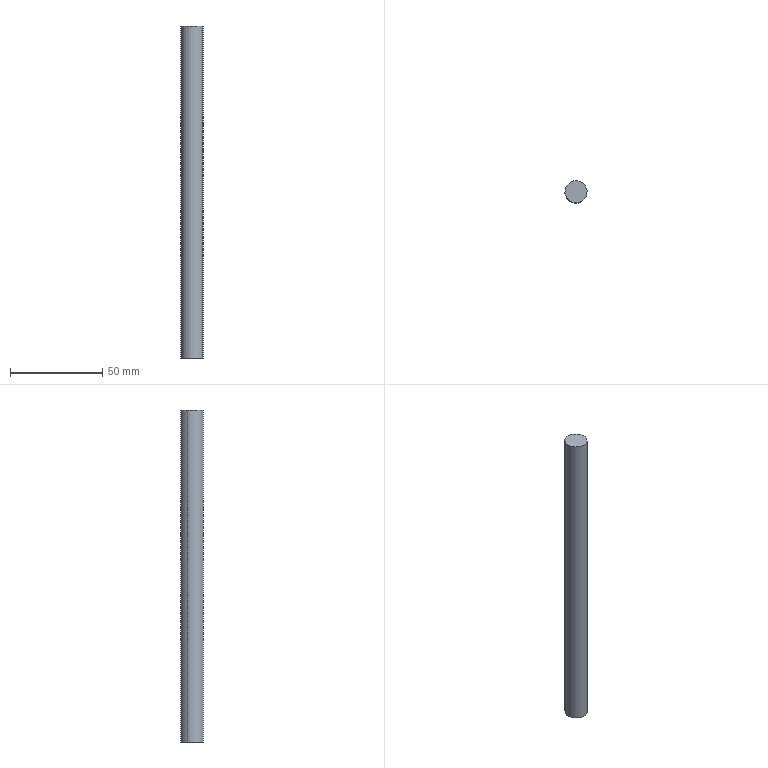Component | SolidWorks | MainAxis-1 | 1 solid | 4 faces | box 12 x 12 x 180 mm | volume 20358 mm3 | cylinder 2 | plane 2 | commonest cylinder face diameters 12 x2
build123d program:
from build123d import *

# Parameters (mm, degrees)
BOSS_EXTRUDE1_DEPTH      = 100
BOSS_EXTRUDE1_DEPTH_BACK = 80
SKETCH1_R                = 6


with BuildPart() as part:
    # Sketch1 → Boss-Extrude1 (new, two sides: drawn at the far end of the back side and taken through both)
    with BuildSketch(Plane.XY.offset(-BOSS_EXTRUDE1_DEPTH_BACK)):
        with Locations((-45, 0)):
            Circle(SKETCH1_R)
    extrude(amount=BOSS_EXTRUDE1_DEPTH + BOSS_EXTRUDE1_DEPTH_BACK)


solid = part.part

# Placed as in the assembly
solid = solid.moved(Location((-24.375, -67.172, 27.182), (0, 0, 0)))
STEP:
#1=CARTESIAN_POINT('',(-2.948,-2.551,-2.079));
#2=VERTEX_POINT('',#1);
#3=CARTESIAN_POINT('',(-2.514,-2.738,-2.079));
#4=VERTEX_POINT('',#3);
#5=CARTESIAN_POINT('',(-2.731,-2.645,-2.079));
#6=DIRECTION('',(-0.,0.,1.));
#7=DIRECTION('',(-0.918,0.3966,0.));
#8=AXIS2_PLACEMENT_3D('',#5,#6,#7);
#9=CIRCLE('',#8,0.2362);
#10=EDGE_CURVE('',#2,#4,#9,.T.);
#11=ORIENTED_EDGE('',*,*,#10,.T.);
#12=CARTESIAN_POINT('',(-2.514,-2.738,5.007));
#13=VERTEX_POINT('',#12);
#14=CARTESIAN_POINT('',(-2.514,-2.738,-2.079));
#15=DIRECTION('',(-0.,0.,1.));
#16=VECTOR('',#15,39.37);
#17=LINE('',#14,#16);
#18=EDGE_CURVE('',#4,#13,#17,.T.);
#19=ORIENTED_EDGE('',*,*,#18,.T.);
#20=CARTESIAN_POINT('',(-2.948,-2.551,5.007));
#21=VERTEX_POINT('',#20);
#22=CARTESIAN_POINT('',(-2.731,-2.645,5.007));
#23=DIRECTION('',(-0.,0.,1.));
#24=DIRECTION('',(-0.918,0.3966,0.));
#25=AXIS2_PLACEMENT_3D('',#22,#23,#24);
#26=CIRCLE('',#25,0.2362);
#27=EDGE_CURVE('',#21,#13,#26,.T.);
#28=ORIENTED_EDGE('',*,*,#27,.F.);
#29=CARTESIAN_POINT('',(-2.948,-2.551,-2.079));
#30=DIRECTION('',(-0.,0.,1.));
#31=VECTOR('',#30,39.37);
#32=LINE('',#29,#31);
#33=EDGE_CURVE('',#2,#21,#32,.T.);
#34=ORIENTED_EDGE('',*,*,#33,.F.);
#35=EDGE_LOOP('',(#11,#19,#28,#34));
#36=FACE_OUTER_BOUND('',#35,.T.);
#37=CARTESIAN_POINT('',(-2.731,-2.645,-2.079));
#38=DIRECTION('',(-0.,0.,1.));
#39=DIRECTION('',(-0.918,0.3966,0.));
#40=AXIS2_PLACEMENT_3D('',#37,#38,#39);
#41=CYLINDRICAL_SURFACE('',#40,0.2362);
#42=ADVANCED_FACE('',(#36),#41,.T.);
#43=ORIENTED_EDGE('',*,*,#18,.F.);
#44=CARTESIAN_POINT('',(-2.731,-2.645,-2.079));
#45=DIRECTION('',(-0.,0.,1.));
#46=DIRECTION('',(-0.918,0.3966,0.));
#47=AXIS2_PLACEMENT_3D('',#44,#45,#46);
#48=CIRCLE('',#47,0.2362);
#49=EDGE_CURVE('',#4,#2,#48,.T.);
#50=ORIENTED_EDGE('',*,*,#49,.T.);
#51=ORIENTED_EDGE('',*,*,#33,.T.);
#52=CARTESIAN_POINT('',(-2.731,-2.645,5.007));
#53=DIRECTION('',(-0.,0.,1.));
#54=DIRECTION('',(-0.918,0.3966,0.));
#55=AXIS2_PLACEMENT_3D('',#52,#53,#54);
#56=CIRCLE('',#55,0.2362);
#57=EDGE_CURVE('',#13,#21,#56,.T.);
#58=ORIENTED_EDGE('',*,*,#57,.F.);
#59=EDGE_LOOP('',(#43,#50,#51,#58));
#60=FACE_OUTER_BOUND('',#59,.T.);
#61=CARTESIAN_POINT('',(-2.731,-2.645,-2.079));
#62=DIRECTION('',(-0.,0.,1.));
#63=DIRECTION('',(-0.918,0.3966,0.));
#64=AXIS2_PLACEMENT_3D('',#61,#62,#63);
#65=CYLINDRICAL_SURFACE('',#64,0.2362);
#66=ADVANCED_FACE('',(#60),#65,.T.);
#67=ORIENTED_EDGE('',*,*,#10,.F.);
#68=ORIENTED_EDGE('',*,*,#49,.F.);
#69=EDGE_LOOP('',(#67,#68));
#70=FACE_OUTER_BOUND('',#69,.T.);
#71=CARTESIAN_POINT('',(-2.731,-2.645,-2.079));
#72=DIRECTION('',(-0.,0.,1.));
#73=DIRECTION('',(-0.918,0.3966,-0.));
#74=AXIS2_PLACEMENT_3D('',#71,#72,#73);
#75=PLANE('',#74);
#76=ADVANCED_FACE('',(#70),#75,.F.);
#77=ORIENTED_EDGE('',*,*,#27,.T.);
#78=ORIENTED_EDGE('',*,*,#57,.T.);
#79=EDGE_LOOP('',(#77,#78));
#80=FACE_OUTER_BOUND('',#79,.T.);
#81=CARTESIAN_POINT('',(-2.731,-2.645,5.007));
#82=DIRECTION('',(-0.,0.,1.));
#83=DIRECTION('',(-0.918,0.3966,-0.));
#84=AXIS2_PLACEMENT_3D('',#81,#82,#83);
#85=PLANE('',#84);
#86=ADVANCED_FACE('',(#80),#85,.T.);
#87=CLOSED_SHELL('',(#42,#66,#76,#86));
#88=MANIFOLD_SOLID_BREP('',#87);
#89=CARTESIAN_POINT('',(0.,0.,0.));
#90=DIRECTION('',(0.,0.,1.));
#91=DIRECTION('',(1.,0.,0.));
#92=AXIS2_PLACEMENT_3D('',#89,#90,#91);
#93=(LENGTH_UNIT()NAMED_UNIT(*)SI_UNIT($,.METRE.));
#94=LENGTH_MEASURE_WITH_UNIT(LENGTH_MEASURE(0.0254),#93);
#95=DIMENSIONAL_EXPONENTS(1.,0.,0.,0.,0.,0.,0.);
#96=(CONVERSION_BASED_UNIT('',#94)LENGTH_UNIT()NAMED_UNIT(#95));
#97=UNCERTAINTY_MEASURE_WITH_UNIT(LENGTH_MEASURE(0.00001),#96,'','');
#98=(NAMED_UNIT(*)PLANE_ANGLE_UNIT()SI_UNIT($,.RADIAN.));
#99=(NAMED_UNIT(*)SI_UNIT($,.STERADIAN.)SOLID_ANGLE_UNIT());
#100=(GEOMETRIC_REPRESENTATION_CONTEXT(3)GLOBAL_UNCERTAINTY_ASSIGNED_CONTEXT((#97))GLOBAL_UNIT_ASSIGNED_CONTEXT((#96,#98,#99))REPRESENTATION_CONTEXT('',''));
#101=ADVANCED_BREP_SHAPE_REPRESENTATION('',(#88,#92),#100);
#102=COLOUR_RGB('',0.7922,0.8196,0.9333);
#103=FILL_AREA_STYLE_COLOUR('',#102);
#104=FILL_AREA_STYLE('',(#103));
#105=SURFACE_STYLE_FILL_AREA(#104);
#106=SURFACE_SIDE_STYLE('',(#105));
#107=SURFACE_STYLE_USAGE(.BOTH.,#106);
#108=PRESENTATION_STYLE_ASSIGNMENT((#107));
#109=STYLED_ITEM('',(#108),#88);
#110=(LENGTH_UNIT()NAMED_UNIT(*)SI_UNIT($,.METRE.));
#111=LENGTH_MEASURE_WITH_UNIT(LENGTH_MEASURE(0.0254),#110);
#112=DIMENSIONAL_EXPONENTS(1.,0.,0.,0.,0.,0.,0.);
#113=(CONVERSION_BASED_UNIT('',#111)LENGTH_UNIT()NAMED_UNIT(#112));
#114=UNCERTAINTY_MEASURE_WITH_UNIT(LENGTH_MEASURE(0.00001),#113,'','');
#115=(NAMED_UNIT(*)PLANE_ANGLE_UNIT()SI_UNIT($,.RADIAN.));
#116=(NAMED_UNIT(*)SI_UNIT($,.STERADIAN.)SOLID_ANGLE_UNIT());
#117=(GEOMETRIC_REPRESENTATION_CONTEXT(3)GLOBAL_UNCERTAINTY_ASSIGNED_CONTEXT((#114))GLOBAL_UNIT_ASSIGNED_CONTEXT((#113,#115,#116))REPRESENTATION_CONTEXT('',''));
#118=MECHANICAL_DESIGN_GEOMETRIC_PRESENTATION_REPRESENTATION('',(#109),#117);
#119=PRESENTATION_LAYER_ASSIGNMENT('','',(#109));